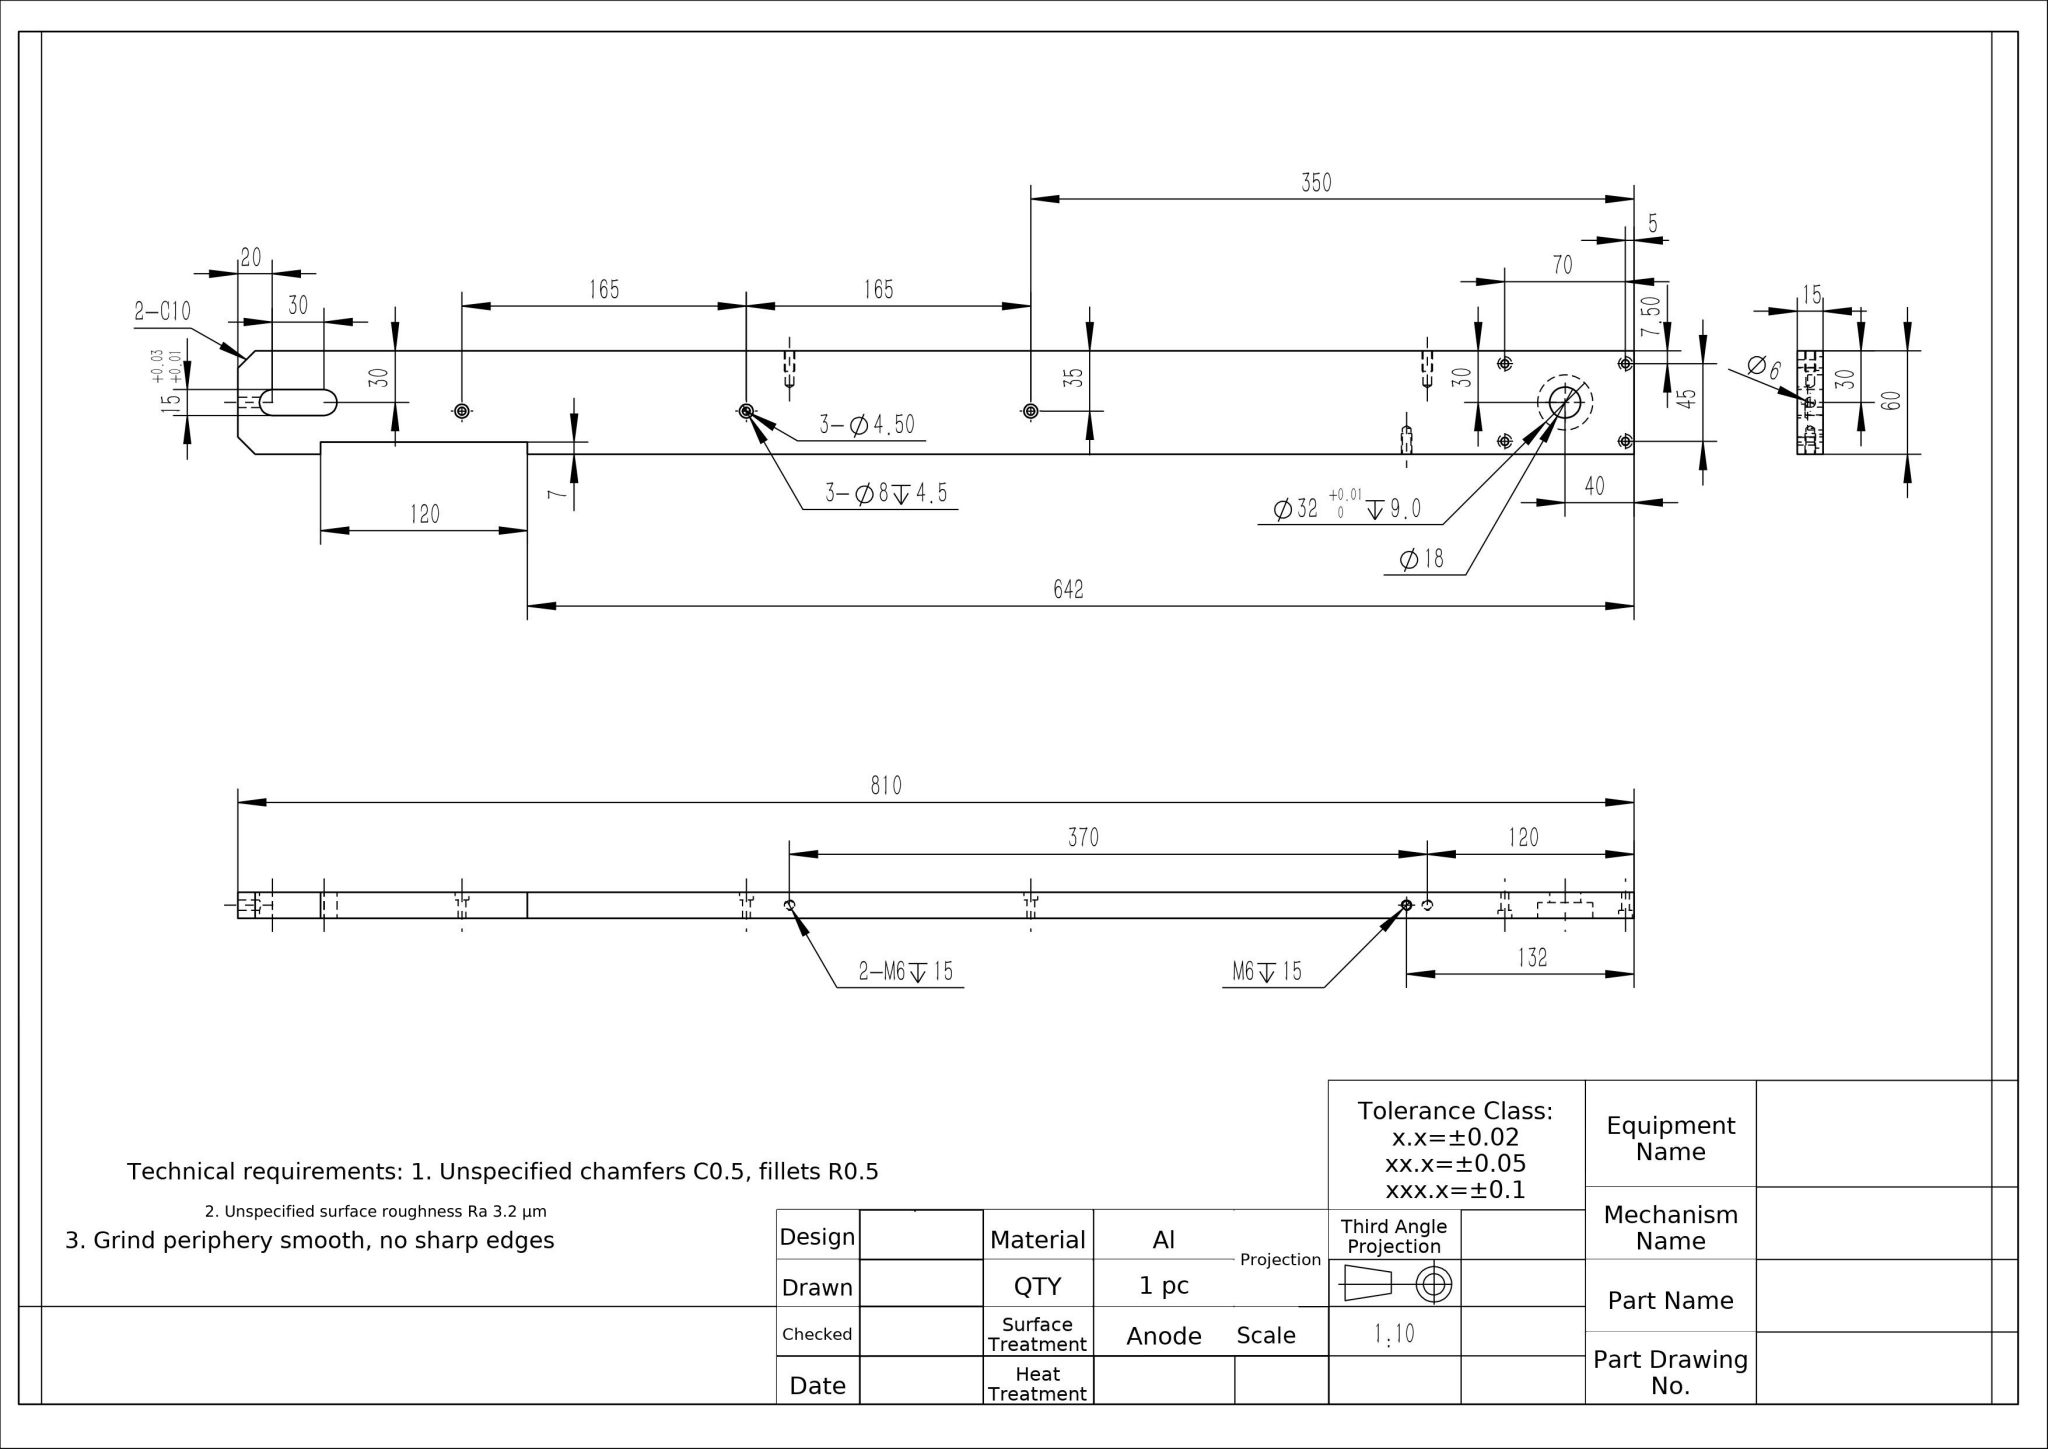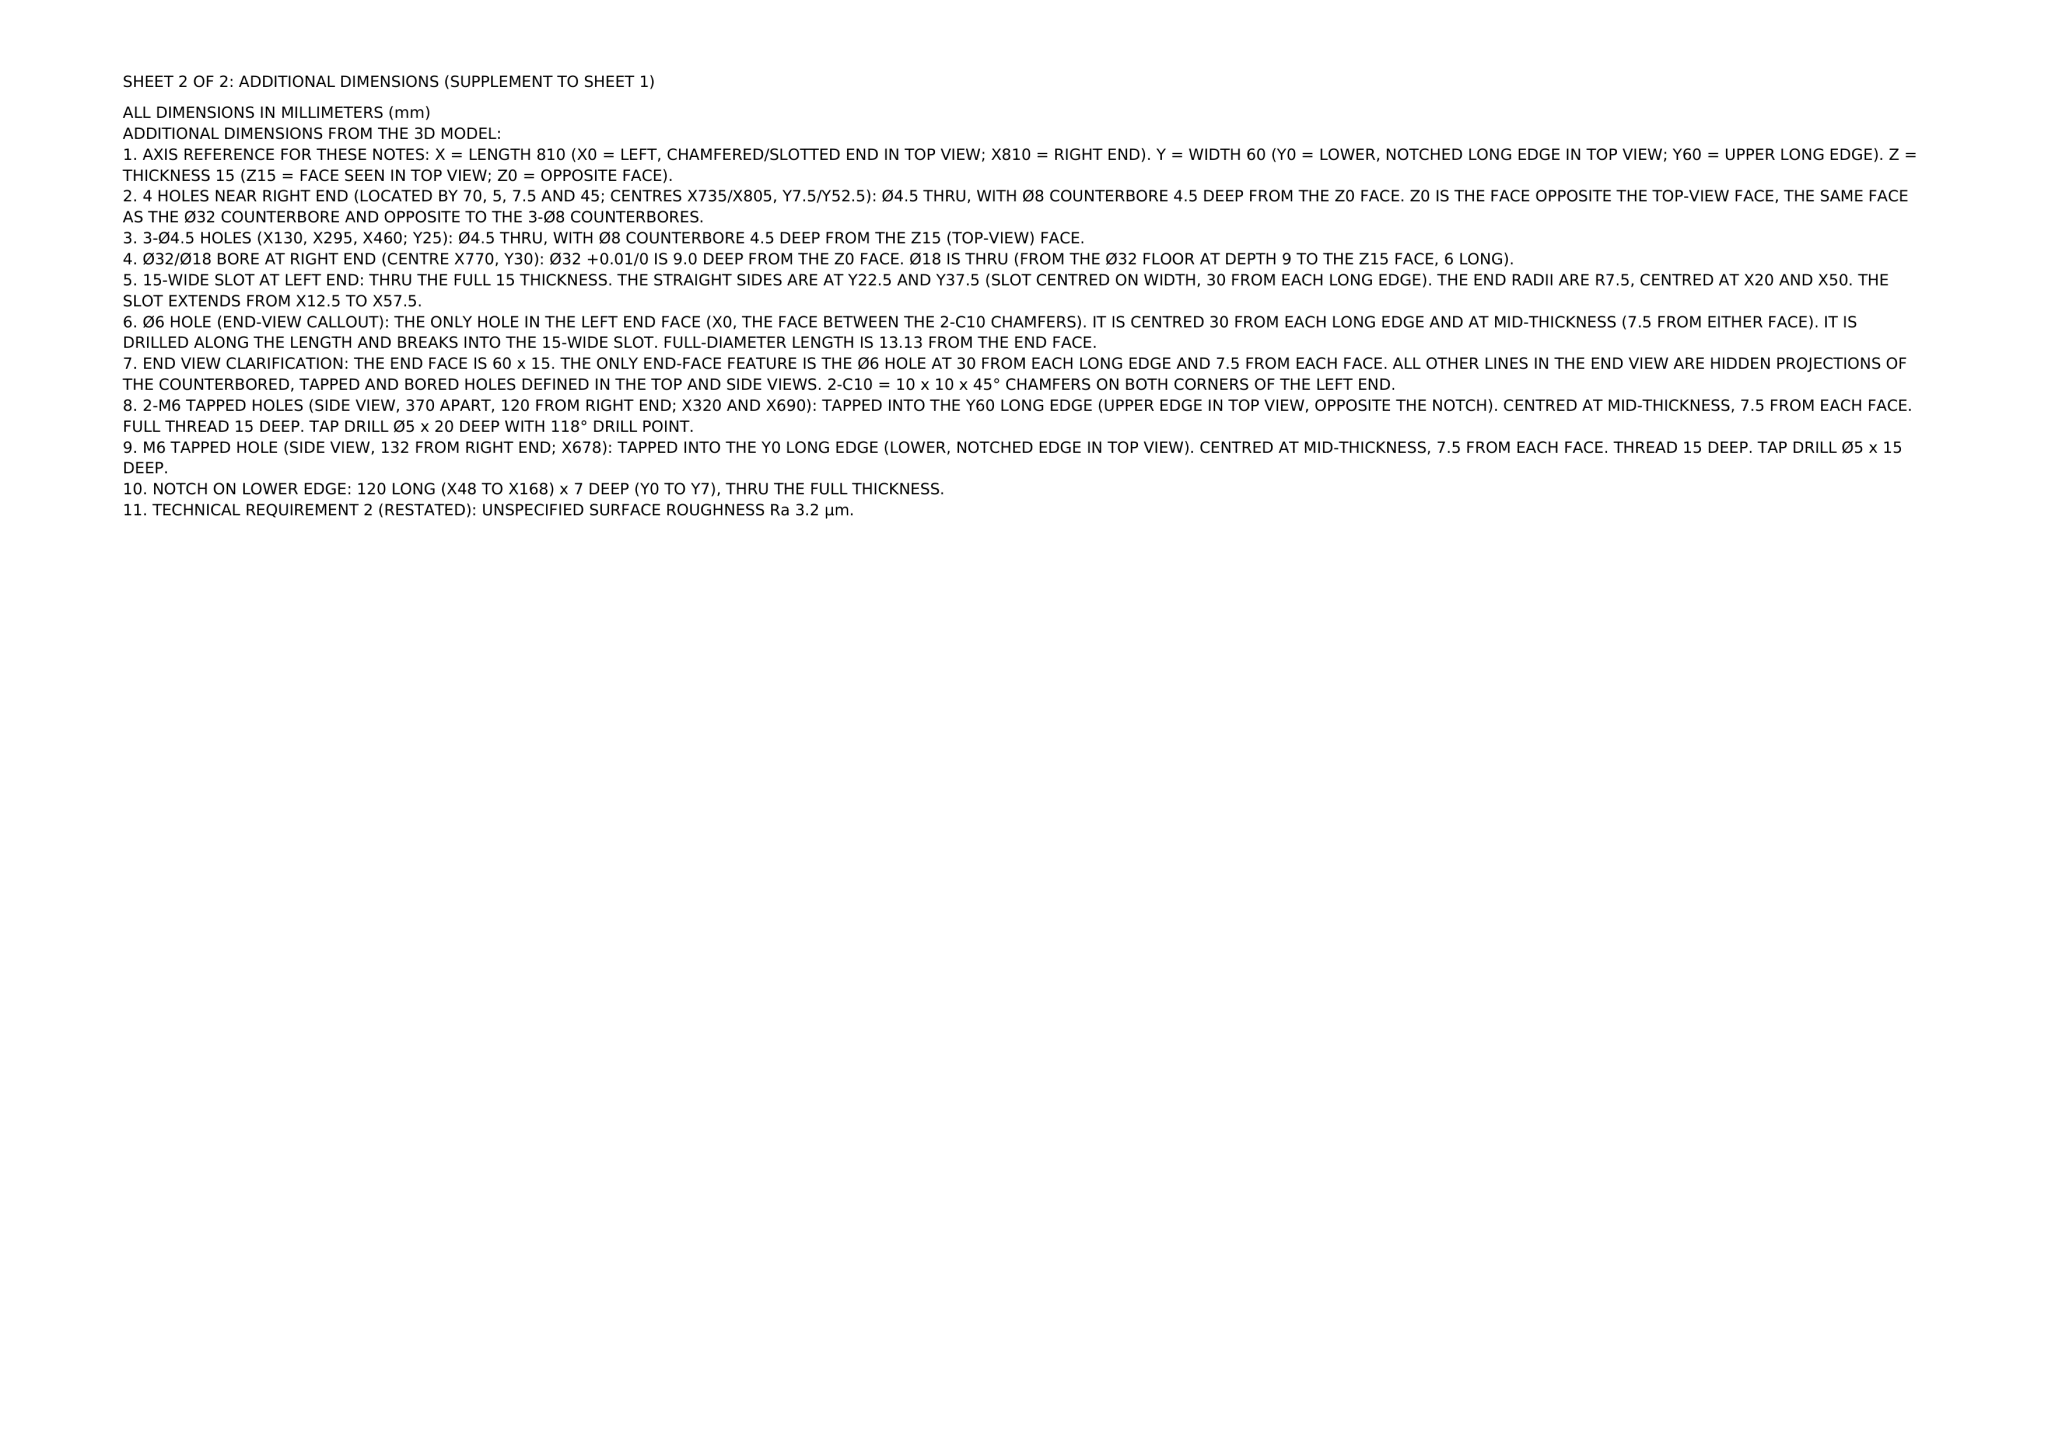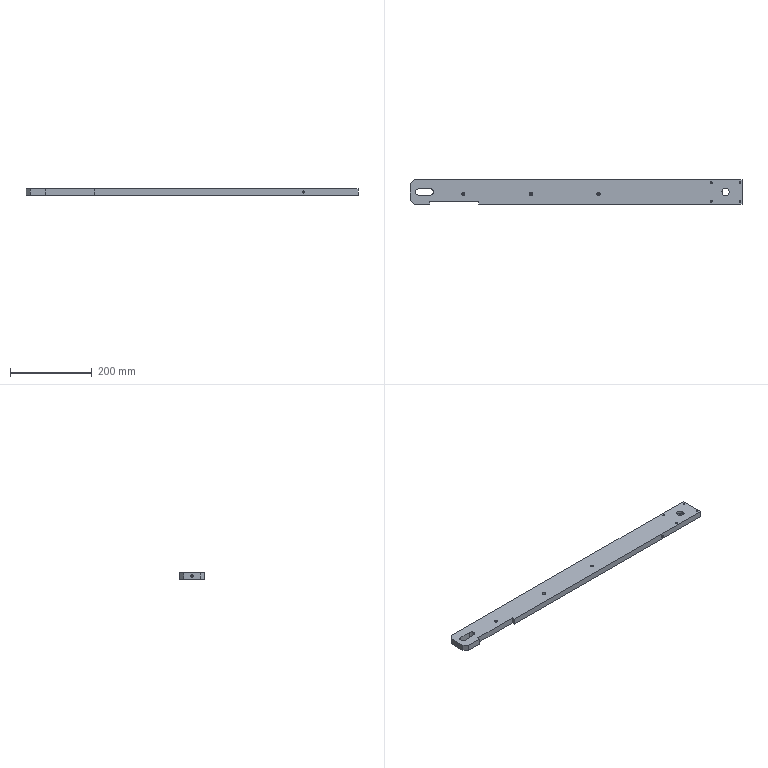Part | NX | mm | Stepped Notched Mounting Bar | 1 solid | 71 faces | box 810 x 60 x 15 mm | volume 692515 mm3 | cylinder 43 | plane 22 | cone 6 | commonest cylinder face diameters 8 x14 4.5 x14 5 x6 15 x3 6 x2 32 x2 18 x2